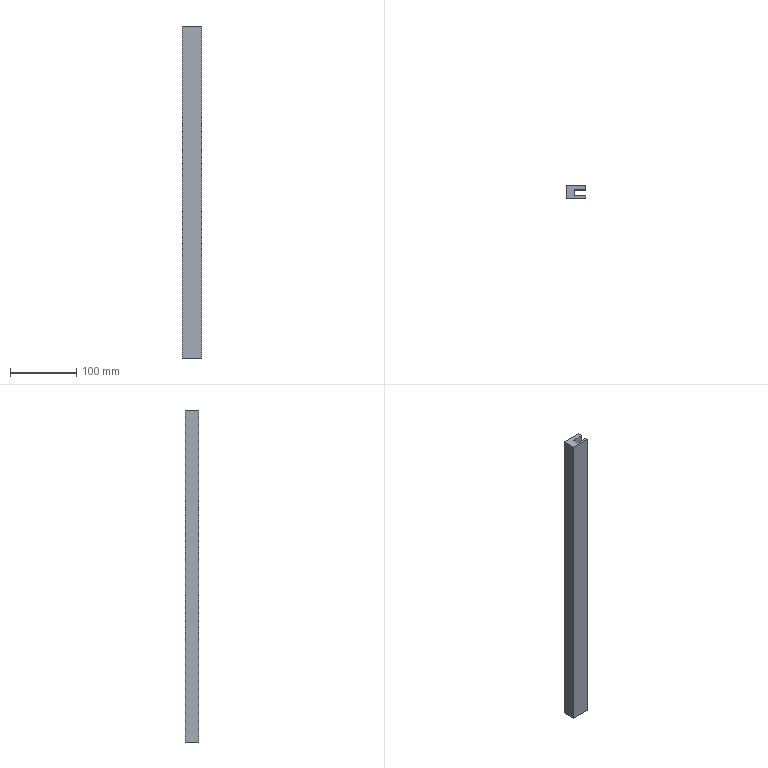Component | NX | SLIDE_CHANNEL_2 | 1 solid | 10 faces | box 30 x 20 x 500 mm | volume 219723 mm3 | plane 10
STEP:
#1=CARTESIAN_POINT('',(0.,0.,0.));
#2=DIRECTION('',(0.,0.,1.));
#3=DIRECTION('',(1.,0.,0.));
#4=AXIS2_PLACEMENT_3D('',#1,#2,#3);
#5=CARTESIAN_POINT('',(-310.,-376.752,150.));
#6=VERTEX_POINT('',#5);
#7=CARTESIAN_POINT('',(-310.,-376.752,650.));
#8=VERTEX_POINT('',#7);
#9=CARTESIAN_POINT('',(-310.,-376.752,650.));
#10=DIRECTION('',(-0.,0.,1.));
#11=VECTOR('',#10,1.);
#12=LINE('',#9,#11);
#13=CARTESIAN_POINT('',(-310.,-390.,650.));
#14=DIRECTION('',(1.,0.,0.));
#15=DIRECTION('',(0.,0.,-1.));
#16=AXIS2_PLACEMENT_3D('',#13,#14,#15);
#17=PLANE('',#16);
#18=CARTESIAN_POINT('',(0.,13.248));
#19=DIRECTION('',(-1.,0.));
#20=VECTOR('',#19,1.);
#21=LINE('',#18,#20);
#22=(GEOMETRIC_REPRESENTATION_CONTEXT(2)PARAMETRIC_REPRESENTATION_CONTEXT()REPRESENTATION_CONTEXT('',''));
#23=DEFINITIONAL_REPRESENTATION('',(#21),#22);
#24=PCURVE('',#17,#23);
#25=CARTESIAN_POINT('',(-321.907,-376.752,670.));
#26=DIRECTION('',(0.,1.,0.));
#27=DIRECTION('',(0.,0.,1.));
#28=AXIS2_PLACEMENT_3D('',#25,#26,#27);
#29=PLANE('',#28);
#30=CARTESIAN_POINT('',(-20.,11.907));
#31=DIRECTION('',(1.,-0.));
#32=VECTOR('',#31,1.);
#33=LINE('',#30,#32);
#34=(GEOMETRIC_REPRESENTATION_CONTEXT(2)PARAMETRIC_REPRESENTATION_CONTEXT()REPRESENTATION_CONTEXT('',''));
#35=DEFINITIONAL_REPRESENTATION('',(#33),#34);
#36=PCURVE('',#29,#35);
#37=SURFACE_CURVE('',#12,(#24,#36),.PCURVE_S1.);
#38=EDGE_CURVE('',#6,#8,#37,.T.);
#39=ORIENTED_EDGE('',*,*,#38,.F.);
#40=CARTESIAN_POINT('',(-310.,-370.,150.));
#41=VERTEX_POINT('',#40);
#42=CARTESIAN_POINT('',(-310.,-390.,150.));
#43=DIRECTION('',(0.,1.,0.));
#44=VECTOR('',#43,1.);
#45=LINE('',#42,#44);
#46=CARTESIAN_POINT('',(500.,0.));
#47=DIRECTION('',(0.,1.));
#48=VECTOR('',#47,1.);
#49=LINE('',#46,#48);
#50=(GEOMETRIC_REPRESENTATION_CONTEXT(2)PARAMETRIC_REPRESENTATION_CONTEXT()REPRESENTATION_CONTEXT('',''));
#51=DEFINITIONAL_REPRESENTATION('',(#49),#50);
#52=PCURVE('',#17,#51);
#53=CARTESIAN_POINT('',(-310.,-390.,150.));
#54=DIRECTION('',(0.,0.,-1.));
#55=DIRECTION('',(-1.,0.,0.));
#56=AXIS2_PLACEMENT_3D('',#53,#54,#55);
#57=PLANE('',#56);
#58=CARTESIAN_POINT('',(0.,0.));
#59=DIRECTION('',(0.,1.));
#60=VECTOR('',#59,1.);
#61=LINE('',#58,#60);
#62=(GEOMETRIC_REPRESENTATION_CONTEXT(2)PARAMETRIC_REPRESENTATION_CONTEXT()REPRESENTATION_CONTEXT('',''));
#63=DEFINITIONAL_REPRESENTATION('',(#61),#62);
#64=PCURVE('',#57,#63);
#65=SURFACE_CURVE('',#45,(#52,#64),.PCURVE_S1.);
#66=EDGE_CURVE('',#6,#41,#65,.T.);
#67=ORIENTED_EDGE('',*,*,#66,.T.);
#68=CARTESIAN_POINT('',(-310.,-370.,650.));
#69=VERTEX_POINT('',#68);
#70=CARTESIAN_POINT('',(-310.,-370.,650.));
#71=DIRECTION('',(0.,0.,-1.));
#72=VECTOR('',#71,1.);
#73=LINE('',#70,#72);
#74=CARTESIAN_POINT('',(0.,20.));
#75=DIRECTION('',(1.,0.));
#76=VECTOR('',#75,1.);
#77=LINE('',#74,#76);
#78=(GEOMETRIC_REPRESENTATION_CONTEXT(2)PARAMETRIC_REPRESENTATION_CONTEXT()REPRESENTATION_CONTEXT('',''));
#79=DEFINITIONAL_REPRESENTATION('',(#77),#78);
#80=PCURVE('',#17,#79);
#81=CARTESIAN_POINT('',(0.,-370.,0.));
#82=DIRECTION('',(0.,1.,0.));
#83=DIRECTION('',(0.,0.,1.));
#84=AXIS2_PLACEMENT_3D('',#81,#82,#83);
#85=PLANE('',#84);
#86=CARTESIAN_POINT('',(650.,-310.));
#87=DIRECTION('',(-1.,0.));
#88=VECTOR('',#87,1.);
#89=LINE('',#86,#88);
#90=(GEOMETRIC_REPRESENTATION_CONTEXT(2)PARAMETRIC_REPRESENTATION_CONTEXT()REPRESENTATION_CONTEXT('',''));
#91=DEFINITIONAL_REPRESENTATION('',(#89),#90);
#92=PCURVE('',#85,#91);
#93=SURFACE_CURVE('',#73,(#80,#92),.PCURVE_S1.);
#94=EDGE_CURVE('',#69,#41,#93,.T.);
#95=ORIENTED_EDGE('',*,*,#94,.F.);
#96=CARTESIAN_POINT('',(-310.,-390.,650.));
#97=DIRECTION('',(0.,1.,0.));
#98=VECTOR('',#97,1.);
#99=LINE('',#96,#98);
#100=CARTESIAN_POINT('',(0.,0.));
#101=DIRECTION('',(0.,1.));
#102=VECTOR('',#101,1.);
#103=LINE('',#100,#102);
#104=(GEOMETRIC_REPRESENTATION_CONTEXT(2)PARAMETRIC_REPRESENTATION_CONTEXT()REPRESENTATION_CONTEXT('',''));
#105=DEFINITIONAL_REPRESENTATION('',(#103),#104);
#106=PCURVE('',#17,#105);
#107=CARTESIAN_POINT('',(-340.,-390.,650.));
#108=DIRECTION('',(0.,0.,1.));
#109=DIRECTION('',(1.,0.,0.));
#110=AXIS2_PLACEMENT_3D('',#107,#108,#109);
#111=PLANE('',#110);
#112=CARTESIAN_POINT('',(30.,0.));
#113=DIRECTION('',(0.,1.));
#114=VECTOR('',#113,1.);
#115=LINE('',#112,#114);
#116=(GEOMETRIC_REPRESENTATION_CONTEXT(2)PARAMETRIC_REPRESENTATION_CONTEXT()REPRESENTATION_CONTEXT('',''));
#117=DEFINITIONAL_REPRESENTATION('',(#115),#116);
#118=PCURVE('',#111,#117);
#119=SURFACE_CURVE('',#99,(#106,#118),.PCURVE_S1.);
#120=EDGE_CURVE('',#8,#69,#119,.T.);
#121=ORIENTED_EDGE('',*,*,#120,.F.);
#122=EDGE_LOOP('',(#39,#67,#95,#121));
#123=FACE_BOUND('',#122,.T.);
#124=ADVANCED_FACE('',(#123),#17,.T.);
#125=CARTESIAN_POINT('',(-340.,-370.,150.));
#126=VERTEX_POINT('',#125);
#127=CARTESIAN_POINT('',(-340.,-370.,650.));
#128=VERTEX_POINT('',#127);
#129=CARTESIAN_POINT('',(-340.,-370.,150.));
#130=DIRECTION('',(-0.,0.,1.));
#131=VECTOR('',#130,1.);
#132=LINE('',#129,#131);
#133=CARTESIAN_POINT('',(-340.,-390.,150.));
#134=DIRECTION('',(-1.,0.,-0.));
#135=DIRECTION('',(-0.,0.,1.));
#136=AXIS2_PLACEMENT_3D('',#133,#134,#135);
#137=PLANE('',#136);
#138=CARTESIAN_POINT('',(0.,20.));
#139=DIRECTION('',(1.,0.));
#140=VECTOR('',#139,1.);
#141=LINE('',#138,#140);
#142=(GEOMETRIC_REPRESENTATION_CONTEXT(2)PARAMETRIC_REPRESENTATION_CONTEXT()REPRESENTATION_CONTEXT('',''));
#143=DEFINITIONAL_REPRESENTATION('',(#141),#142);
#144=PCURVE('',#137,#143);
#145=CARTESIAN_POINT('',(150.,-340.));
#146=DIRECTION('',(1.,-0.));
#147=VECTOR('',#146,1.);
#148=LINE('',#145,#147);
#149=(GEOMETRIC_REPRESENTATION_CONTEXT(2)PARAMETRIC_REPRESENTATION_CONTEXT()REPRESENTATION_CONTEXT('',''));
#150=DEFINITIONAL_REPRESENTATION('',(#148),#149);
#151=PCURVE('',#85,#150);
#152=SURFACE_CURVE('',#132,(#144,#151),.PCURVE_S1.);
#153=EDGE_CURVE('',#126,#128,#152,.T.);
#154=ORIENTED_EDGE('',*,*,#153,.F.);
#155=CARTESIAN_POINT('',(-340.,-390.,150.));
#156=VERTEX_POINT('',#155);
#157=CARTESIAN_POINT('',(-340.,-390.,150.));
#158=DIRECTION('',(0.,1.,0.));
#159=VECTOR('',#158,1.);
#160=LINE('',#157,#159);
#161=CARTESIAN_POINT('',(0.,0.));
#162=DIRECTION('',(0.,1.));
#163=VECTOR('',#162,1.);
#164=LINE('',#161,#163);
#165=(GEOMETRIC_REPRESENTATION_CONTEXT(2)PARAMETRIC_REPRESENTATION_CONTEXT()REPRESENTATION_CONTEXT('',''));
#166=DEFINITIONAL_REPRESENTATION('',(#164),#165);
#167=PCURVE('',#137,#166);
#168=CARTESIAN_POINT('',(30.,0.));
#169=DIRECTION('',(0.,1.));
#170=VECTOR('',#169,1.);
#171=LINE('',#168,#170);
#172=(GEOMETRIC_REPRESENTATION_CONTEXT(2)PARAMETRIC_REPRESENTATION_CONTEXT()REPRESENTATION_CONTEXT('',''));
#173=DEFINITIONAL_REPRESENTATION('',(#171),#172);
#174=PCURVE('',#57,#173);
#175=SURFACE_CURVE('',#160,(#167,#174),.PCURVE_S1.);
#176=EDGE_CURVE('',#156,#126,#175,.T.);
#177=ORIENTED_EDGE('',*,*,#176,.F.);
#178=CARTESIAN_POINT('',(-340.,-390.,650.));
#179=VERTEX_POINT('',#178);
#180=CARTESIAN_POINT('',(-340.,-390.,150.));
#181=DIRECTION('',(-0.,0.,1.));
#182=VECTOR('',#181,1.);
#183=LINE('',#180,#182);
#184=CARTESIAN_POINT('',(0.,0.));
#185=DIRECTION('',(1.,0.));
#186=VECTOR('',#185,1.);
#187=LINE('',#184,#186);
#188=(GEOMETRIC_REPRESENTATION_CONTEXT(2)PARAMETRIC_REPRESENTATION_CONTEXT()REPRESENTATION_CONTEXT('',''));
#189=DEFINITIONAL_REPRESENTATION('',(#187),#188);
#190=PCURVE('',#137,#189);
#191=CARTESIAN_POINT('',(0.,-390.,0.));
#192=DIRECTION('',(0.,1.,0.));
#193=DIRECTION('',(0.,0.,1.));
#194=AXIS2_PLACEMENT_3D('',#191,#192,#193);
#195=PLANE('',#194);
#196=CARTESIAN_POINT('',(150.,-340.));
#197=DIRECTION('',(1.,-0.));
#198=VECTOR('',#197,1.);
#199=LINE('',#196,#198);
#200=(GEOMETRIC_REPRESENTATION_CONTEXT(2)PARAMETRIC_REPRESENTATION_CONTEXT()REPRESENTATION_CONTEXT('',''));
#201=DEFINITIONAL_REPRESENTATION('',(#199),#200);
#202=PCURVE('',#195,#201);
#203=SURFACE_CURVE('',#183,(#190,#202),.PCURVE_S1.);
#204=EDGE_CURVE('',#156,#179,#203,.T.);
#205=ORIENTED_EDGE('',*,*,#204,.T.);
#206=CARTESIAN_POINT('',(-340.,-390.,650.));
#207=DIRECTION('',(0.,1.,0.));
#208=VECTOR('',#207,1.);
#209=LINE('',#206,#208);
#210=CARTESIAN_POINT('',(500.,0.));
#211=DIRECTION('',(0.,1.));
#212=VECTOR('',#211,1.);
#213=LINE('',#210,#212);
#214=(GEOMETRIC_REPRESENTATION_CONTEXT(2)PARAMETRIC_REPRESENTATION_CONTEXT()REPRESENTATION_CONTEXT('',''));
#215=DEFINITIONAL_REPRESENTATION('',(#213),#214);
#216=PCURVE('',#137,#215);
#217=CARTESIAN_POINT('',(0.,0.));
#218=DIRECTION('',(0.,1.));
#219=VECTOR('',#218,1.);
#220=LINE('',#217,#219);
#221=(GEOMETRIC_REPRESENTATION_CONTEXT(2)PARAMETRIC_REPRESENTATION_CONTEXT()REPRESENTATION_CONTEXT('',''));
#222=DEFINITIONAL_REPRESENTATION('',(#220),#221);
#223=PCURVE('',#111,#222);
#224=SURFACE_CURVE('',#209,(#216,#223),.PCURVE_S1.);
#225=EDGE_CURVE('',#179,#128,#224,.T.);
#226=ORIENTED_EDGE('',*,*,#225,.T.);
#227=EDGE_LOOP('',(#154,#177,#205,#226));
#228=FACE_BOUND('',#227,.T.);
#229=ADVANCED_FACE('',(#228),#137,.T.);
#230=CARTESIAN_POINT('',(-326.907,-376.752,650.));
#231=VERTEX_POINT('',#230);
#232=CARTESIAN_POINT('',(-340.,-376.752,650.));
#233=DIRECTION('',(-1.,0.,0.));
#234=VECTOR('',#233,1.);
#235=LINE('',#232,#234);
#236=CARTESIAN_POINT('',(0.,13.248));
#237=DIRECTION('',(-1.,0.));
#238=VECTOR('',#237,1.);
#239=LINE('',#236,#238);
#240=(GEOMETRIC_REPRESENTATION_CONTEXT(2)PARAMETRIC_REPRESENTATION_CONTEXT()REPRESENTATION_CONTEXT('',''));
#241=DEFINITIONAL_REPRESENTATION('',(#239),#240);
#242=PCURVE('',#111,#241);
#243=CARTESIAN_POINT('',(-20.,-18.093));
#244=DIRECTION('',(0.,-1.));
#245=VECTOR('',#244,1.);
#246=LINE('',#243,#245);
#247=(GEOMETRIC_REPRESENTATION_CONTEXT(2)PARAMETRIC_REPRESENTATION_CONTEXT()REPRESENTATION_CONTEXT('',''));
#248=DEFINITIONAL_REPRESENTATION('',(#246),#247);
#249=PCURVE('',#29,#248);
#250=SURFACE_CURVE('',#235,(#242,#249),.PCURVE_S1.);
#251=EDGE_CURVE('',#8,#231,#250,.T.);
#252=ORIENTED_EDGE('',*,*,#251,.F.);
#253=ORIENTED_EDGE('',*,*,#120,.T.);
#254=CARTESIAN_POINT('',(-340.,-370.,650.));
#255=DIRECTION('',(1.,0.,0.));
#256=VECTOR('',#255,1.);
#257=LINE('',#254,#256);
#258=CARTESIAN_POINT('',(0.,20.));
#259=DIRECTION('',(1.,0.));
#260=VECTOR('',#259,1.);
#261=LINE('',#258,#260);
#262=(GEOMETRIC_REPRESENTATION_CONTEXT(2)PARAMETRIC_REPRESENTATION_CONTEXT()REPRESENTATION_CONTEXT('',''));
#263=DEFINITIONAL_REPRESENTATION('',(#261),#262);
#264=PCURVE('',#111,#263);
#265=CARTESIAN_POINT('',(650.,-340.));
#266=DIRECTION('',(0.,1.));
#267=VECTOR('',#266,1.);
#268=LINE('',#265,#267);
#269=(GEOMETRIC_REPRESENTATION_CONTEXT(2)PARAMETRIC_REPRESENTATION_CONTEXT()REPRESENTATION_CONTEXT('',''));
#270=DEFINITIONAL_REPRESENTATION('',(#268),#269);
#271=PCURVE('',#85,#270);
#272=SURFACE_CURVE('',#257,(#264,#271),.PCURVE_S1.);
#273=EDGE_CURVE('',#128,#69,#272,.T.);
#274=ORIENTED_EDGE('',*,*,#273,.F.);
#275=ORIENTED_EDGE('',*,*,#225,.F.);
#276=CARTESIAN_POINT('',(-310.,-390.,650.));
#277=VERTEX_POINT('',#276);
#278=CARTESIAN_POINT('',(-340.,-390.,650.));
#279=DIRECTION('',(1.,0.,0.));
#280=VECTOR('',#279,1.);
#281=LINE('',#278,#280);
#282=CARTESIAN_POINT('',(0.,0.));
#283=DIRECTION('',(1.,0.));
#284=VECTOR('',#283,1.);
#285=LINE('',#282,#284);
#286=(GEOMETRIC_REPRESENTATION_CONTEXT(2)PARAMETRIC_REPRESENTATION_CONTEXT()REPRESENTATION_CONTEXT('',''));
#287=DEFINITIONAL_REPRESENTATION('',(#285),#286);
#288=PCURVE('',#111,#287);
#289=CARTESIAN_POINT('',(650.,-340.));
#290=DIRECTION('',(0.,1.));
#291=VECTOR('',#290,1.);
#292=LINE('',#289,#291);
#293=(GEOMETRIC_REPRESENTATION_CONTEXT(2)PARAMETRIC_REPRESENTATION_CONTEXT()REPRESENTATION_CONTEXT('',''));
#294=DEFINITIONAL_REPRESENTATION('',(#292),#293);
#295=PCURVE('',#195,#294);
#296=SURFACE_CURVE('',#281,(#288,#295),.PCURVE_S1.);
#297=EDGE_CURVE('',#179,#277,#296,.T.);
#298=ORIENTED_EDGE('',*,*,#297,.T.);
#299=CARTESIAN_POINT('',(-310.,-386.248,650.));
#300=VERTEX_POINT('',#299);
#301=CARTESIAN_POINT('',(-310.,-390.,650.));
#302=DIRECTION('',(0.,1.,0.));
#303=VECTOR('',#302,1.);
#304=LINE('',#301,#303);
#305=CARTESIAN_POINT('',(30.,0.));
#306=DIRECTION('',(0.,1.));
#307=VECTOR('',#306,1.);
#308=LINE('',#305,#307);
#309=(GEOMETRIC_REPRESENTATION_CONTEXT(2)PARAMETRIC_REPRESENTATION_CONTEXT()REPRESENTATION_CONTEXT('',''));
#310=DEFINITIONAL_REPRESENTATION('',(#308),#309);
#311=PCURVE('',#111,#310);
#312=CARTESIAN_POINT('',(-310.,-390.,650.));
#313=DIRECTION('',(1.,0.,0.));
#314=DIRECTION('',(0.,0.,-1.));
#315=AXIS2_PLACEMENT_3D('',#312,#313,#314);
#316=PLANE('',#315);
#317=CARTESIAN_POINT('',(0.,0.));
#318=DIRECTION('',(0.,1.));
#319=VECTOR('',#318,1.);
#320=LINE('',#317,#319);
#321=(GEOMETRIC_REPRESENTATION_CONTEXT(2)PARAMETRIC_REPRESENTATION_CONTEXT()REPRESENTATION_CONTEXT('',''));
#322=DEFINITIONAL_REPRESENTATION('',(#320),#321);
#323=PCURVE('',#316,#322);
#324=SURFACE_CURVE('',#304,(#311,#323),.PCURVE_S1.);
#325=EDGE_CURVE('',#277,#300,#324,.T.);
#326=ORIENTED_EDGE('',*,*,#325,.T.);
#327=CARTESIAN_POINT('',(-326.907,-386.248,650.));
#328=VERTEX_POINT('',#327);
#329=CARTESIAN_POINT('',(-340.,-386.248,650.));
#330=DIRECTION('',(1.,0.,0.));
#331=VECTOR('',#330,1.);
#332=LINE('',#329,#331);
#333=CARTESIAN_POINT('',(0.,3.752));
#334=DIRECTION('',(1.,0.));
#335=VECTOR('',#334,1.);
#336=LINE('',#333,#335);
#337=(GEOMETRIC_REPRESENTATION_CONTEXT(2)PARAMETRIC_REPRESENTATION_CONTEXT()REPRESENTATION_CONTEXT('',''));
#338=DEFINITIONAL_REPRESENTATION('',(#336),#337);
#339=PCURVE('',#111,#338);
#340=CARTESIAN_POINT('',(-303.536,-386.248,670.));
#341=DIRECTION('',(0.,-1.,0.));
#342=DIRECTION('',(0.,0.,-1.));
#343=AXIS2_PLACEMENT_3D('',#340,#341,#342);
#344=PLANE('',#343);
#345=CARTESIAN_POINT('',(20.,-36.464));
#346=DIRECTION('',(0.,1.));
#347=VECTOR('',#346,1.);
#348=LINE('',#345,#347);
#349=(GEOMETRIC_REPRESENTATION_CONTEXT(2)PARAMETRIC_REPRESENTATION_CONTEXT()REPRESENTATION_CONTEXT('',''));
#350=DEFINITIONAL_REPRESENTATION('',(#348),#349);
#351=PCURVE('',#344,#350);
#352=SURFACE_CURVE('',#332,(#339,#351),.PCURVE_S1.);
#353=EDGE_CURVE('',#328,#300,#352,.T.);
#354=ORIENTED_EDGE('',*,*,#353,.F.);
#355=CARTESIAN_POINT('',(-326.907,-390.,650.));
#356=DIRECTION('',(0.,-1.,0.));
#357=VECTOR('',#356,1.);
#358=LINE('',#355,#357);
#359=CARTESIAN_POINT('',(13.093,0.));
#360=DIRECTION('',(0.,-1.));
#361=VECTOR('',#360,1.);
#362=LINE('',#359,#361);
#363=(GEOMETRIC_REPRESENTATION_CONTEXT(2)PARAMETRIC_REPRESENTATION_CONTEXT()REPRESENTATION_CONTEXT('',''));
#364=DEFINITIONAL_REPRESENTATION('',(#362),#363);
#365=PCURVE('',#111,#364);
#366=CARTESIAN_POINT('',(-326.907,-386.248,670.));
#367=DIRECTION('',(-1.,0.,0.));
#368=DIRECTION('',(0.,0.,1.));
#369=AXIS2_PLACEMENT_3D('',#366,#367,#368);
#370=PLANE('',#369);
#371=CARTESIAN_POINT('',(-20.,-3.752));
#372=DIRECTION('',(0.,-1.));
#373=VECTOR('',#372,1.);
#374=LINE('',#371,#373);
#375=(GEOMETRIC_REPRESENTATION_CONTEXT(2)PARAMETRIC_REPRESENTATION_CONTEXT()REPRESENTATION_CONTEXT('',''));
#376=DEFINITIONAL_REPRESENTATION('',(#374),#375);
#377=PCURVE('',#370,#376);
#378=SURFACE_CURVE('',#358,(#365,#377),.PCURVE_S1.);
#379=EDGE_CURVE('',#231,#328,#378,.T.);
#380=ORIENTED_EDGE('',*,*,#379,.F.);
#381=EDGE_LOOP('',(#252,#253,#274,#275,#298,#326,#354,#380));
#382=FACE_BOUND('',#381,.T.);
#383=ADVANCED_FACE('',(#382),#111,.T.);
#384=CARTESIAN_POINT('',(-310.,-386.248,150.));
#385=VERTEX_POINT('',#384);
#386=CARTESIAN_POINT('',(-310.,-386.248,650.));
#387=DIRECTION('',(0.,0.,-1.));
#388=VECTOR('',#387,1.);
#389=LINE('',#386,#388);
#390=CARTESIAN_POINT('',(0.,3.752));
#391=DIRECTION('',(1.,0.));
#392=VECTOR('',#391,1.);
#393=LINE('',#390,#392);
#394=(GEOMETRIC_REPRESENTATION_CONTEXT(2)PARAMETRIC_REPRESENTATION_CONTEXT()REPRESENTATION_CONTEXT('',''));
#395=DEFINITIONAL_REPRESENTATION('',(#393),#394);
#396=PCURVE('',#316,#395);
#397=CARTESIAN_POINT('',(20.,-6.464));
#398=DIRECTION('',(1.,0.));
#399=VECTOR('',#398,1.);
#400=LINE('',#397,#399);
#401=(GEOMETRIC_REPRESENTATION_CONTEXT(2)PARAMETRIC_REPRESENTATION_CONTEXT()REPRESENTATION_CONTEXT('',''));
#402=DEFINITIONAL_REPRESENTATION('',(#400),#401);
#403=PCURVE('',#344,#402);
#404=SURFACE_CURVE('',#389,(#396,#403),.PCURVE_S1.);
#405=EDGE_CURVE('',#300,#385,#404,.T.);
#406=ORIENTED_EDGE('',*,*,#405,.F.);
#407=ORIENTED_EDGE('',*,*,#325,.F.);
#408=CARTESIAN_POINT('',(-310.,-390.,150.));
#409=VERTEX_POINT('',#408);
#410=CARTESIAN_POINT('',(-310.,-390.,650.));
#411=DIRECTION('',(0.,0.,-1.));
#412=VECTOR('',#411,1.);
#413=LINE('',#410,#412);
#414=CARTESIAN_POINT('',(0.,0.));
#415=DIRECTION('',(1.,0.));
#416=VECTOR('',#415,1.);
#417=LINE('',#414,#416);
#418=(GEOMETRIC_REPRESENTATION_CONTEXT(2)PARAMETRIC_REPRESENTATION_CONTEXT()REPRESENTATION_CONTEXT('',''));
#419=DEFINITIONAL_REPRESENTATION('',(#417),#418);
#420=PCURVE('',#316,#419);
#421=CARTESIAN_POINT('',(650.,-310.));
#422=DIRECTION('',(-1.,0.));
#423=VECTOR('',#422,1.);
#424=LINE('',#421,#423);
#425=(GEOMETRIC_REPRESENTATION_CONTEXT(2)PARAMETRIC_REPRESENTATION_CONTEXT()REPRESENTATION_CONTEXT('',''));
#426=DEFINITIONAL_REPRESENTATION('',(#424),#425);
#427=PCURVE('',#195,#426);
#428=SURFACE_CURVE('',#413,(#420,#427),.PCURVE_S1.);
#429=EDGE_CURVE('',#277,#409,#428,.T.);
#430=ORIENTED_EDGE('',*,*,#429,.T.);
#431=CARTESIAN_POINT('',(-310.,-390.,150.));
#432=DIRECTION('',(0.,1.,0.));
#433=VECTOR('',#432,1.);
#434=LINE('',#431,#433);
#435=CARTESIAN_POINT('',(500.,0.));
#436=DIRECTION('',(0.,1.));
#437=VECTOR('',#436,1.);
#438=LINE('',#435,#437);
#439=(GEOMETRIC_REPRESENTATION_CONTEXT(2)PARAMETRIC_REPRESENTATION_CONTEXT()REPRESENTATION_CONTEXT('',''));
#440=DEFINITIONAL_REPRESENTATION('',(#438),#439);
#441=PCURVE('',#316,#440);
#442=CARTESIAN_POINT('',(0.,0.));
#443=DIRECTION('',(0.,1.));
#444=VECTOR('',#443,1.);
#445=LINE('',#442,#444);
#446=(GEOMETRIC_REPRESENTATION_CONTEXT(2)PARAMETRIC_REPRESENTATION_CONTEXT()REPRESENTATION_CONTEXT('',''));
#447=DEFINITIONAL_REPRESENTATION('',(#445),#446);
#448=PCURVE('',#57,#447);
#449=SURFACE_CURVE('',#434,(#441,#448),.PCURVE_S1.);
#450=EDGE_CURVE('',#409,#385,#449,.T.);
#451=ORIENTED_EDGE('',*,*,#450,.T.);
#452=EDGE_LOOP('',(#406,#407,#430,#451));
#453=FACE_BOUND('',#452,.T.);
#454=ADVANCED_FACE('',(#453),#316,.T.);
#455=CARTESIAN_POINT('',(-326.907,-376.752,150.));
#456=VERTEX_POINT('',#455);
#457=CARTESIAN_POINT('',(-310.,-376.752,150.));
#458=DIRECTION('',(1.,0.,0.));
#459=VECTOR('',#458,1.);
#460=LINE('',#457,#459);
#461=CARTESIAN_POINT('',(0.,13.248));
#462=DIRECTION('',(-1.,0.));
#463=VECTOR('',#462,1.);
#464=LINE('',#461,#463);
#465=(GEOMETRIC_REPRESENTATION_CONTEXT(2)PARAMETRIC_REPRESENTATION_CONTEXT()REPRESENTATION_CONTEXT('',''));
#466=DEFINITIONAL_REPRESENTATION('',(#464),#465);
#467=PCURVE('',#57,#466);
#468=CARTESIAN_POINT('',(-520.,11.907));
#469=DIRECTION('',(0.,1.));
#470=VECTOR('',#469,1.);
#471=LINE('',#468,#470);
#472=(GEOMETRIC_REPRESENTATION_CONTEXT(2)PARAMETRIC_REPRESENTATION_CONTEXT()REPRESENTATION_CONTEXT('',''));
#473=DEFINITIONAL_REPRESENTATION('',(#471),#472);
#474=PCURVE('',#29,#473);
#475=SURFACE_CURVE('',#460,(#467,#474),.PCURVE_S1.);
#476=EDGE_CURVE('',#456,#6,#475,.T.);
#477=ORIENTED_EDGE('',*,*,#476,.F.);
#478=CARTESIAN_POINT('',(-326.907,-386.248,150.));
#479=VERTEX_POINT('',#478);
#480=CARTESIAN_POINT('',(-326.907,-390.,150.));
#481=DIRECTION('',(0.,1.,0.));
#482=VECTOR('',#481,1.);
#483=LINE('',#480,#482);
#484=CARTESIAN_POINT('',(16.907,0.));
#485=DIRECTION('',(0.,1.));
#486=VECTOR('',#485,1.);
#487=LINE('',#484,#486);
#488=(GEOMETRIC_REPRESENTATION_CONTEXT(2)PARAMETRIC_REPRESENTATION_CONTEXT()REPRESENTATION_CONTEXT('',''));
#489=DEFINITIONAL_REPRESENTATION('',(#487),#488);
#490=PCURVE('',#57,#489);
#491=CARTESIAN_POINT('',(-520.,-3.752));
#492=DIRECTION('',(0.,1.));
#493=VECTOR('',#492,1.);
#494=LINE('',#491,#493);
#495=(GEOMETRIC_REPRESENTATION_CONTEXT(2)PARAMETRIC_REPRESENTATION_CONTEXT()REPRESENTATION_CONTEXT('',''));
#496=DEFINITIONAL_REPRESENTATION('',(#494),#495);
#497=PCURVE('',#370,#496);
#498=SURFACE_CURVE('',#483,(#490,#497),.PCURVE_S1.);
#499=EDGE_CURVE('',#479,#456,#498,.T.);
#500=ORIENTED_EDGE('',*,*,#499,.F.);
#501=CARTESIAN_POINT('',(-310.,-386.248,150.));
#502=DIRECTION('',(-1.,0.,0.));
#503=VECTOR('',#502,1.);
#504=LINE('',#501,#503);
#505=CARTESIAN_POINT('',(0.,3.752));
#506=DIRECTION('',(1.,0.));
#507=VECTOR('',#506,1.);
#508=LINE('',#505,#507);
#509=(GEOMETRIC_REPRESENTATION_CONTEXT(2)PARAMETRIC_REPRESENTATION_CONTEXT()REPRESENTATION_CONTEXT('',''));
#510=DEFINITIONAL_REPRESENTATION('',(#508),#509);
#511=PCURVE('',#57,#510);
#512=CARTESIAN_POINT('',(520.,-6.464));
#513=DIRECTION('',(0.,-1.));
#514=VECTOR('',#513,1.);
#515=LINE('',#512,#514);
#516=(GEOMETRIC_REPRESENTATION_CONTEXT(2)PARAMETRIC_REPRESENTATION_CONTEXT()REPRESENTATION_CONTEXT('',''));
#517=DEFINITIONAL_REPRESENTATION('',(#515),#516);
#518=PCURVE('',#344,#517);
#519=SURFACE_CURVE('',#504,(#511,#518),.PCURVE_S1.);
#520=EDGE_CURVE('',#385,#479,#519,.T.);
#521=ORIENTED_EDGE('',*,*,#520,.F.);
#522=ORIENTED_EDGE('',*,*,#450,.F.);
#523=CARTESIAN_POINT('',(-310.,-390.,150.));
#524=DIRECTION('',(-1.,0.,0.));
#525=VECTOR('',#524,1.);
#526=LINE('',#523,#525);
#527=CARTESIAN_POINT('',(0.,0.));
#528=DIRECTION('',(1.,0.));
#529=VECTOR('',#528,1.);
#530=LINE('',#527,#529);
#531=(GEOMETRIC_REPRESENTATION_CONTEXT(2)PARAMETRIC_REPRESENTATION_CONTEXT()REPRESENTATION_CONTEXT('',''));
#532=DEFINITIONAL_REPRESENTATION('',(#530),#531);
#533=PCURVE('',#57,#532);
#534=CARTESIAN_POINT('',(150.,-310.));
#535=DIRECTION('',(0.,-1.));
#536=VECTOR('',#535,1.);
#537=LINE('',#534,#536);
#538=(GEOMETRIC_REPRESENTATION_CONTEXT(2)PARAMETRIC_REPRESENTATION_CONTEXT()REPRESENTATION_CONTEXT('',''));
#539=DEFINITIONAL_REPRESENTATION('',(#537),#538);
#540=PCURVE('',#195,#539);
#541=SURFACE_CURVE('',#526,(#533,#540),.PCURVE_S1.);
#542=EDGE_CURVE('',#409,#156,#541,.T.);
#543=ORIENTED_EDGE('',*,*,#542,.T.);
#544=ORIENTED_EDGE('',*,*,#176,.T.);
#545=CARTESIAN_POINT('',(-310.,-370.,150.));
#546=DIRECTION('',(-1.,0.,0.));
#547=VECTOR('',#546,1.);
#548=LINE('',#545,#547);
#549=CARTESIAN_POINT('',(0.,20.));
#550=DIRECTION('',(1.,0.));
#551=VECTOR('',#550,1.);
#552=LINE('',#549,#551);
#553=(GEOMETRIC_REPRESENTATION_CONTEXT(2)PARAMETRIC_REPRESENTATION_CONTEXT()REPRESENTATION_CONTEXT('',''));
#554=DEFINITIONAL_REPRESENTATION('',(#552),#553);
#555=PCURVE('',#57,#554);
#556=CARTESIAN_POINT('',(150.,-310.));
#557=DIRECTION('',(0.,-1.));
#558=VECTOR('',#557,1.);
#559=LINE('',#556,#558);
#560=(GEOMETRIC_REPRESENTATION_CONTEXT(2)PARAMETRIC_REPRESENTATION_CONTEXT()REPRESENTATION_CONTEXT('',''));
#561=DEFINITIONAL_REPRESENTATION('',(#559),#560);
#562=PCURVE('',#85,#561);
#563=SURFACE_CURVE('',#548,(#555,#562),.PCURVE_S1.);
#564=EDGE_CURVE('',#41,#126,#563,.T.);
#565=ORIENTED_EDGE('',*,*,#564,.F.);
#566=ORIENTED_EDGE('',*,*,#66,.F.);
#567=EDGE_LOOP('',(#477,#500,#521,#522,#543,#544,#565,#566));
#568=FACE_BOUND('',#567,.T.);
#569=ADVANCED_FACE('',(#568),#57,.T.);
#570=ORIENTED_EDGE('',*,*,#204,.F.);
#571=ORIENTED_EDGE('',*,*,#542,.F.);
#572=ORIENTED_EDGE('',*,*,#429,.F.);
#573=ORIENTED_EDGE('',*,*,#297,.F.);
#574=EDGE_LOOP('',(#570,#571,#572,#573));
#575=FACE_BOUND('',#574,.T.);
#576=ADVANCED_FACE('',(#575),#195,.F.);
#577=ORIENTED_EDGE('',*,*,#153,.T.);
#578=ORIENTED_EDGE('',*,*,#273,.T.);
#579=ORIENTED_EDGE('',*,*,#94,.T.);
#580=ORIENTED_EDGE('',*,*,#564,.T.);
#581=EDGE_LOOP('',(#577,#578,#579,#580));
#582=FACE_BOUND('',#581,.T.);
#583=ADVANCED_FACE('',(#582),#85,.T.);
#584=ORIENTED_EDGE('',*,*,#379,.T.);
#585=CARTESIAN_POINT('',(-326.907,-386.248,670.));
#586=DIRECTION('',(0.,0.,1.));
#587=VECTOR('',#586,1.);
#588=LINE('',#585,#587);
#589=CARTESIAN_POINT('',(0.,0.));
#590=DIRECTION('',(1.,0.));
#591=VECTOR('',#590,1.);
#592=LINE('',#589,#591);
#593=(GEOMETRIC_REPRESENTATION_CONTEXT(2)PARAMETRIC_REPRESENTATION_CONTEXT()REPRESENTATION_CONTEXT('',''));
#594=DEFINITIONAL_REPRESENTATION('',(#592),#593);
#595=PCURVE('',#370,#594);
#596=CARTESIAN_POINT('',(0.,-23.371));
#597=DIRECTION('',(-1.,0.));
#598=VECTOR('',#597,1.);
#599=LINE('',#596,#598);
#600=(GEOMETRIC_REPRESENTATION_CONTEXT(2)PARAMETRIC_REPRESENTATION_CONTEXT()REPRESENTATION_CONTEXT('',''));
#601=DEFINITIONAL_REPRESENTATION('',(#599),#600);
#602=PCURVE('',#344,#601);
#603=SURFACE_CURVE('',#588,(#595,#602),.PCURVE_S1.);
#604=EDGE_CURVE('',#479,#328,#603,.T.);
#605=ORIENTED_EDGE('',*,*,#604,.F.);
#606=ORIENTED_EDGE('',*,*,#499,.T.);
#607=CARTESIAN_POINT('',(-326.907,-376.752,670.));
#608=DIRECTION('',(0.,0.,1.));
#609=VECTOR('',#608,1.);
#610=LINE('',#607,#609);
#611=CARTESIAN_POINT('',(0.,9.496));
#612=DIRECTION('',(1.,0.));
#613=VECTOR('',#612,1.);
#614=LINE('',#611,#613);
#615=(GEOMETRIC_REPRESENTATION_CONTEXT(2)PARAMETRIC_REPRESENTATION_CONTEXT()REPRESENTATION_CONTEXT('',''));
#616=DEFINITIONAL_REPRESENTATION('',(#614),#615);
#617=PCURVE('',#370,#616);
#618=CARTESIAN_POINT('',(0.,-5.));
#619=DIRECTION('',(1.,0.));
#620=VECTOR('',#619,1.);
#621=LINE('',#618,#620);
#622=(GEOMETRIC_REPRESENTATION_CONTEXT(2)PARAMETRIC_REPRESENTATION_CONTEXT()REPRESENTATION_CONTEXT('',''));
#623=DEFINITIONAL_REPRESENTATION('',(#621),#622);
#624=PCURVE('',#29,#623);
#625=SURFACE_CURVE('',#610,(#617,#624),.PCURVE_S1.);
#626=EDGE_CURVE('',#456,#231,#625,.T.);
#627=ORIENTED_EDGE('',*,*,#626,.T.);
#628=EDGE_LOOP('',(#584,#605,#606,#627));
#629=FACE_BOUND('',#628,.T.);
#630=ADVANCED_FACE('',(#629),#370,.F.);
#631=ORIENTED_EDGE('',*,*,#251,.T.);
#632=ORIENTED_EDGE('',*,*,#626,.F.);
#633=ORIENTED_EDGE('',*,*,#476,.T.);
#634=ORIENTED_EDGE('',*,*,#38,.T.);
#635=EDGE_LOOP('',(#631,#632,#633,#634));
#636=FACE_BOUND('',#635,.T.);
#637=ADVANCED_FACE('',(#636),#29,.F.);
#638=ORIENTED_EDGE('',*,*,#353,.T.);
#639=ORIENTED_EDGE('',*,*,#405,.T.);
#640=ORIENTED_EDGE('',*,*,#520,.T.);
#641=ORIENTED_EDGE('',*,*,#604,.T.);
#642=EDGE_LOOP('',(#638,#639,#640,#641));
#643=FACE_BOUND('',#642,.T.);
#644=ADVANCED_FACE('',(#643),#344,.F.);
#645=CLOSED_SHELL('',(#124,#229,#383,#454,#569,#576,#583,#630,#637,#644));
#646=MANIFOLD_SOLID_BREP('',#645);
#647=(LENGTH_UNIT()NAMED_UNIT(*)SI_UNIT(.MILLI.,.METRE.));
#648=UNCERTAINTY_MEASURE_WITH_UNIT(LENGTH_MEASURE(0.0000001),#647,'','');
#649=(NAMED_UNIT(*)PLANE_ANGLE_UNIT()SI_UNIT($,.RADIAN.));
#650=(NAMED_UNIT(*)SI_UNIT($,.STERADIAN.)SOLID_ANGLE_UNIT());
#651=(GEOMETRIC_REPRESENTATION_CONTEXT(3)GLOBAL_UNCERTAINTY_ASSIGNED_CONTEXT((#648))GLOBAL_UNIT_ASSIGNED_CONTEXT((#647,#649,#650))REPRESENTATION_CONTEXT('',''));
#652=ADVANCED_BREP_SHAPE_REPRESENTATION('',(#4,#646),#651);